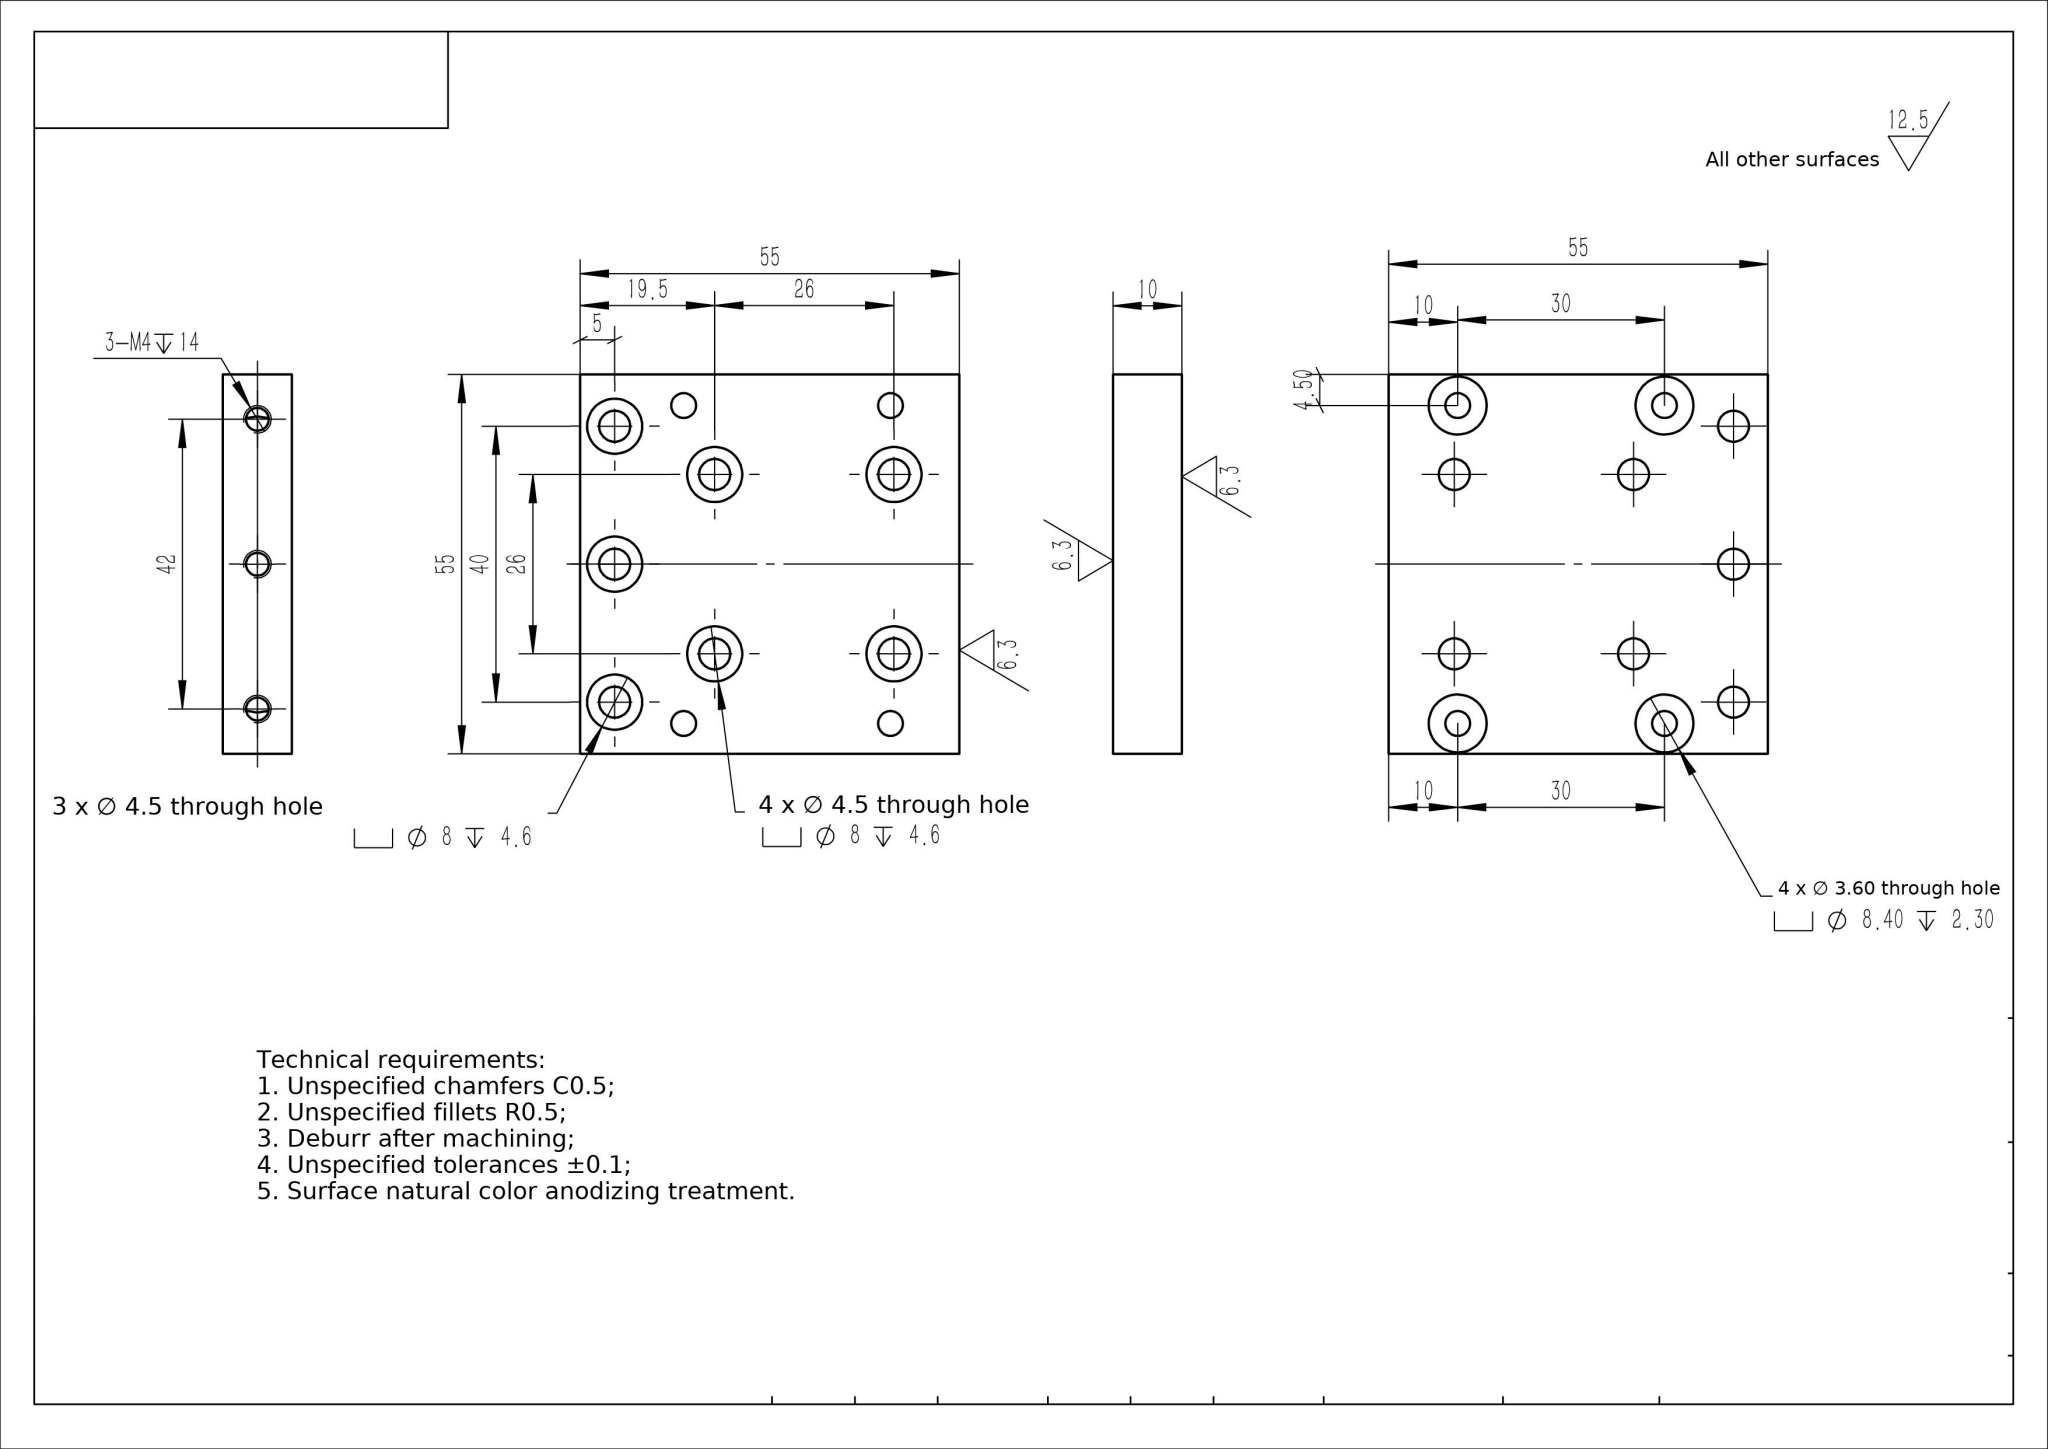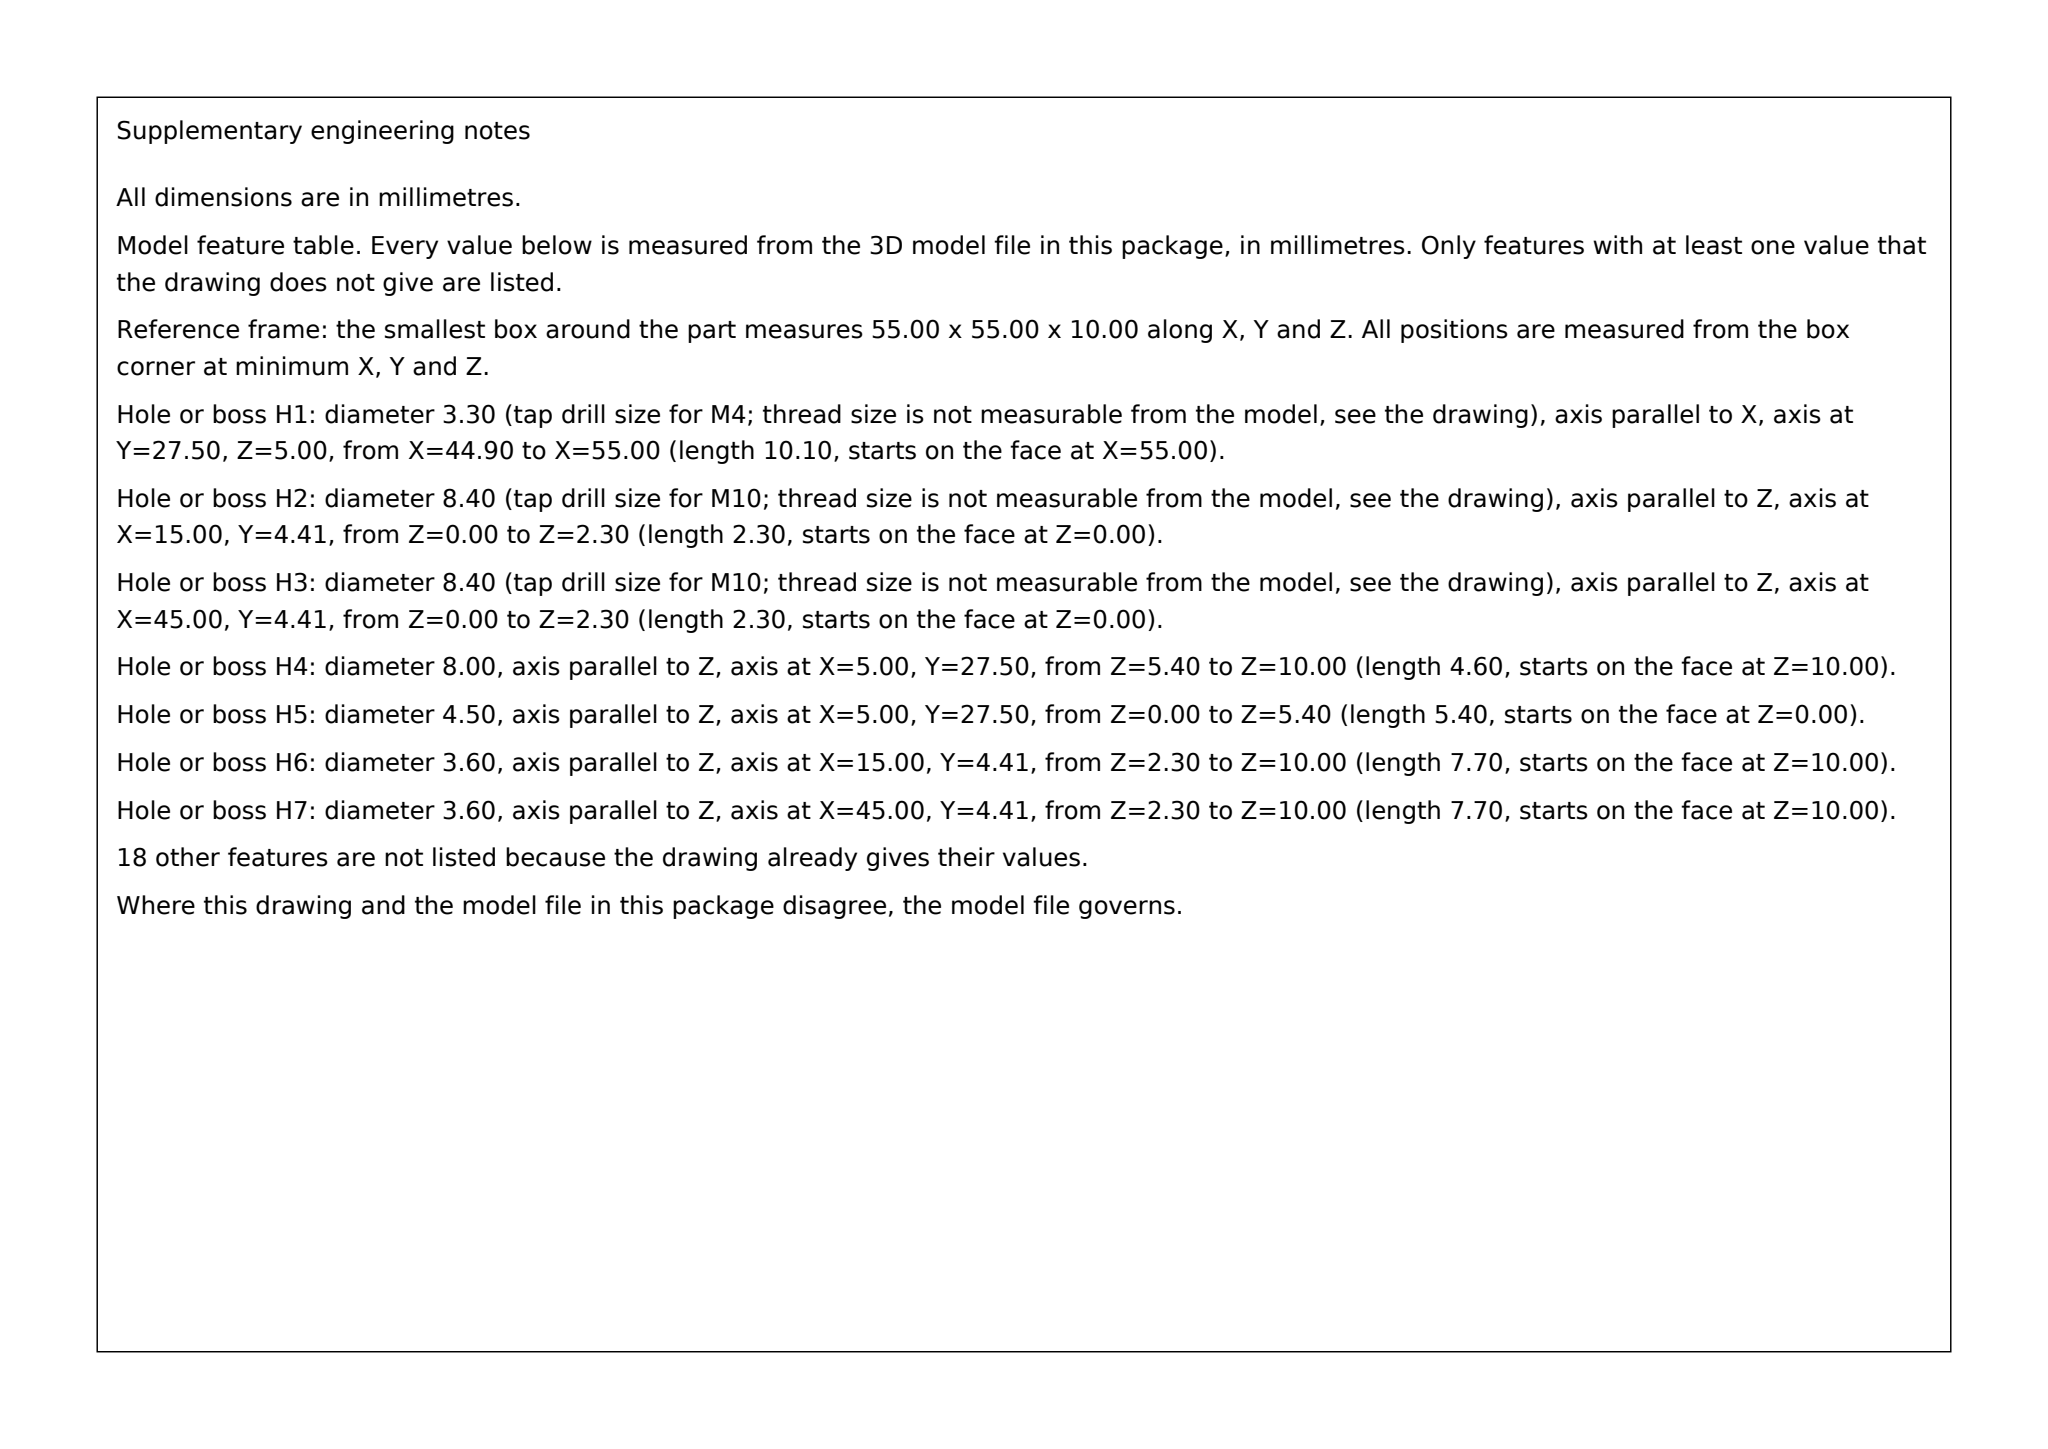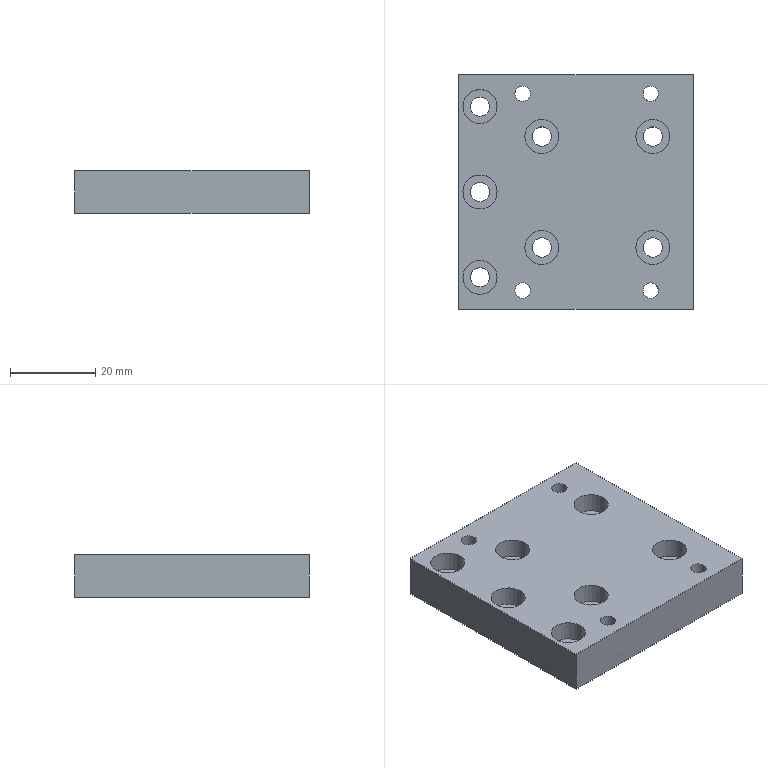Part | SolidWorks | mm | 1 solid | 73 faces | box 55 x 55 x 10 mm | volume 26950 mm3 | cylinder 50 | plane 17 | cone 6 | commonest cylinder face diameters 8 x14 4.5 x14 8.4 x8 3.6 x8 3.3 x6
build123d program:
from build123d import *

# Parameters (mm, degrees)
SKETCH1_W                                           = 55
SKETCH1_H                                           = 55
BOSS_EXTRUDE1_DEPTH                                 = 10
HOLE_SIZE_ACCORDING_TO_HEXAGON_SOCKET_H_D           = 4.5
HOLE_SIZE_ACCORDING_TO_HEXAGON_SOCKET_H_CBORE_D     = 8
HOLE_SIZE_ACCORDING_TO_HEXAGON_SOCKET_H_CBORE_DEPTH = 4.6
HOLE_SIZE_ACCORDING_TO_HEXAGON_SOCK_2_D             = 4.5
HOLE_SIZE_ACCORDING_TO_HEXAGON_SOCK_2_CBORE_D       = 8
HOLE_SIZE_ACCORDING_TO_HEXAGON_SOCK_2_CBORE_DEPTH   = 4.6
M4_TAPPED_HOLE1_D                                   = 3.3
M4_TAPPED_HOLE1_DEPTH                               = 10.1
M4_TAPPED_HOLE1_TIP                                 = 0.9914
M3_HEX_HEAD_MACHINE_SCREW_COUNTERBORE1_D            = 3.6
M3_HEX_HEAD_MACHINE_SCREW_COUNTERBORE1_CBORE_D      = 8.4
M3_HEX_HEAD_MACHINE_SCREW_COUNTERBORE1_CBORE_DEPTH  = 2.3


with BuildPart() as part:
    # Sketch1 → Boss-Extrude1 (new body)
    with BuildSketch(Plane.XY):
        Rectangle(SKETCH1_W, SKETCH1_H)
    extrude(amount=BOSS_EXTRUDE1_DEPTH)

    # Hole Size_ according to_Hexagon Socket H (through all)
    with Locations(Plane.XY.offset(10)):
        with Locations((-22.5, 20), (-22.5, -20), (-22.5, 0)):
            CounterBoreHole(HOLE_SIZE_ACCORDING_TO_HEXAGON_SOCKET_H_D / 2, HOLE_SIZE_ACCORDING_TO_HEXAGON_SOCKET_H_CBORE_D / 2, HOLE_SIZE_ACCORDING_TO_HEXAGON_SOCKET_H_CBORE_DEPTH)

    # Hole Size_ according to_Hexagon Sock 2 (through all)
    with Locations(Plane.XY.offset(10)):
        with Locations((-8, 13), (-8, -13), (18, 13), (18, -13)):
            CounterBoreHole(HOLE_SIZE_ACCORDING_TO_HEXAGON_SOCK_2_D / 2, HOLE_SIZE_ACCORDING_TO_HEXAGON_SOCK_2_CBORE_D / 2, HOLE_SIZE_ACCORDING_TO_HEXAGON_SOCK_2_CBORE_DEPTH)

    # M4 Tapped Hole1
    with Locations(Plane(origin=(27.5, 0, 0), x_dir=(0, 0, -1), z_dir=(1, 0, 0))):
        with Locations((-5, -21), (-5, 21), (-5, 0)):
            Hole(M4_TAPPED_HOLE1_D / 2, depth=M4_TAPPED_HOLE1_DEPTH)
            with Locations((0, 0, -(M4_TAPPED_HOLE1_DEPTH + M4_TAPPED_HOLE1_TIP / 2))):  # 118° drill point
                Cone(0, M4_TAPPED_HOLE1_D / 2, M4_TAPPED_HOLE1_TIP, mode=Mode.SUBTRACT)

    # M3 Hex Head Machine Screw Counterbore1 (through all)
    with Locations(Plane(origin=(0, 0, 0), x_dir=(-1, 0, 0), z_dir=(0, 0, -1))):
        with Locations((-17.5, 23), (12.5, 23), (-17.5, -23.094), (12.5, -23.094)):
            CounterBoreHole(M3_HEX_HEAD_MACHINE_SCREW_COUNTERBORE1_D / 2, M3_HEX_HEAD_MACHINE_SCREW_COUNTERBORE1_CBORE_D / 2, M3_HEX_HEAD_MACHINE_SCREW_COUNTERBORE1_CBORE_DEPTH)


solid = part.part